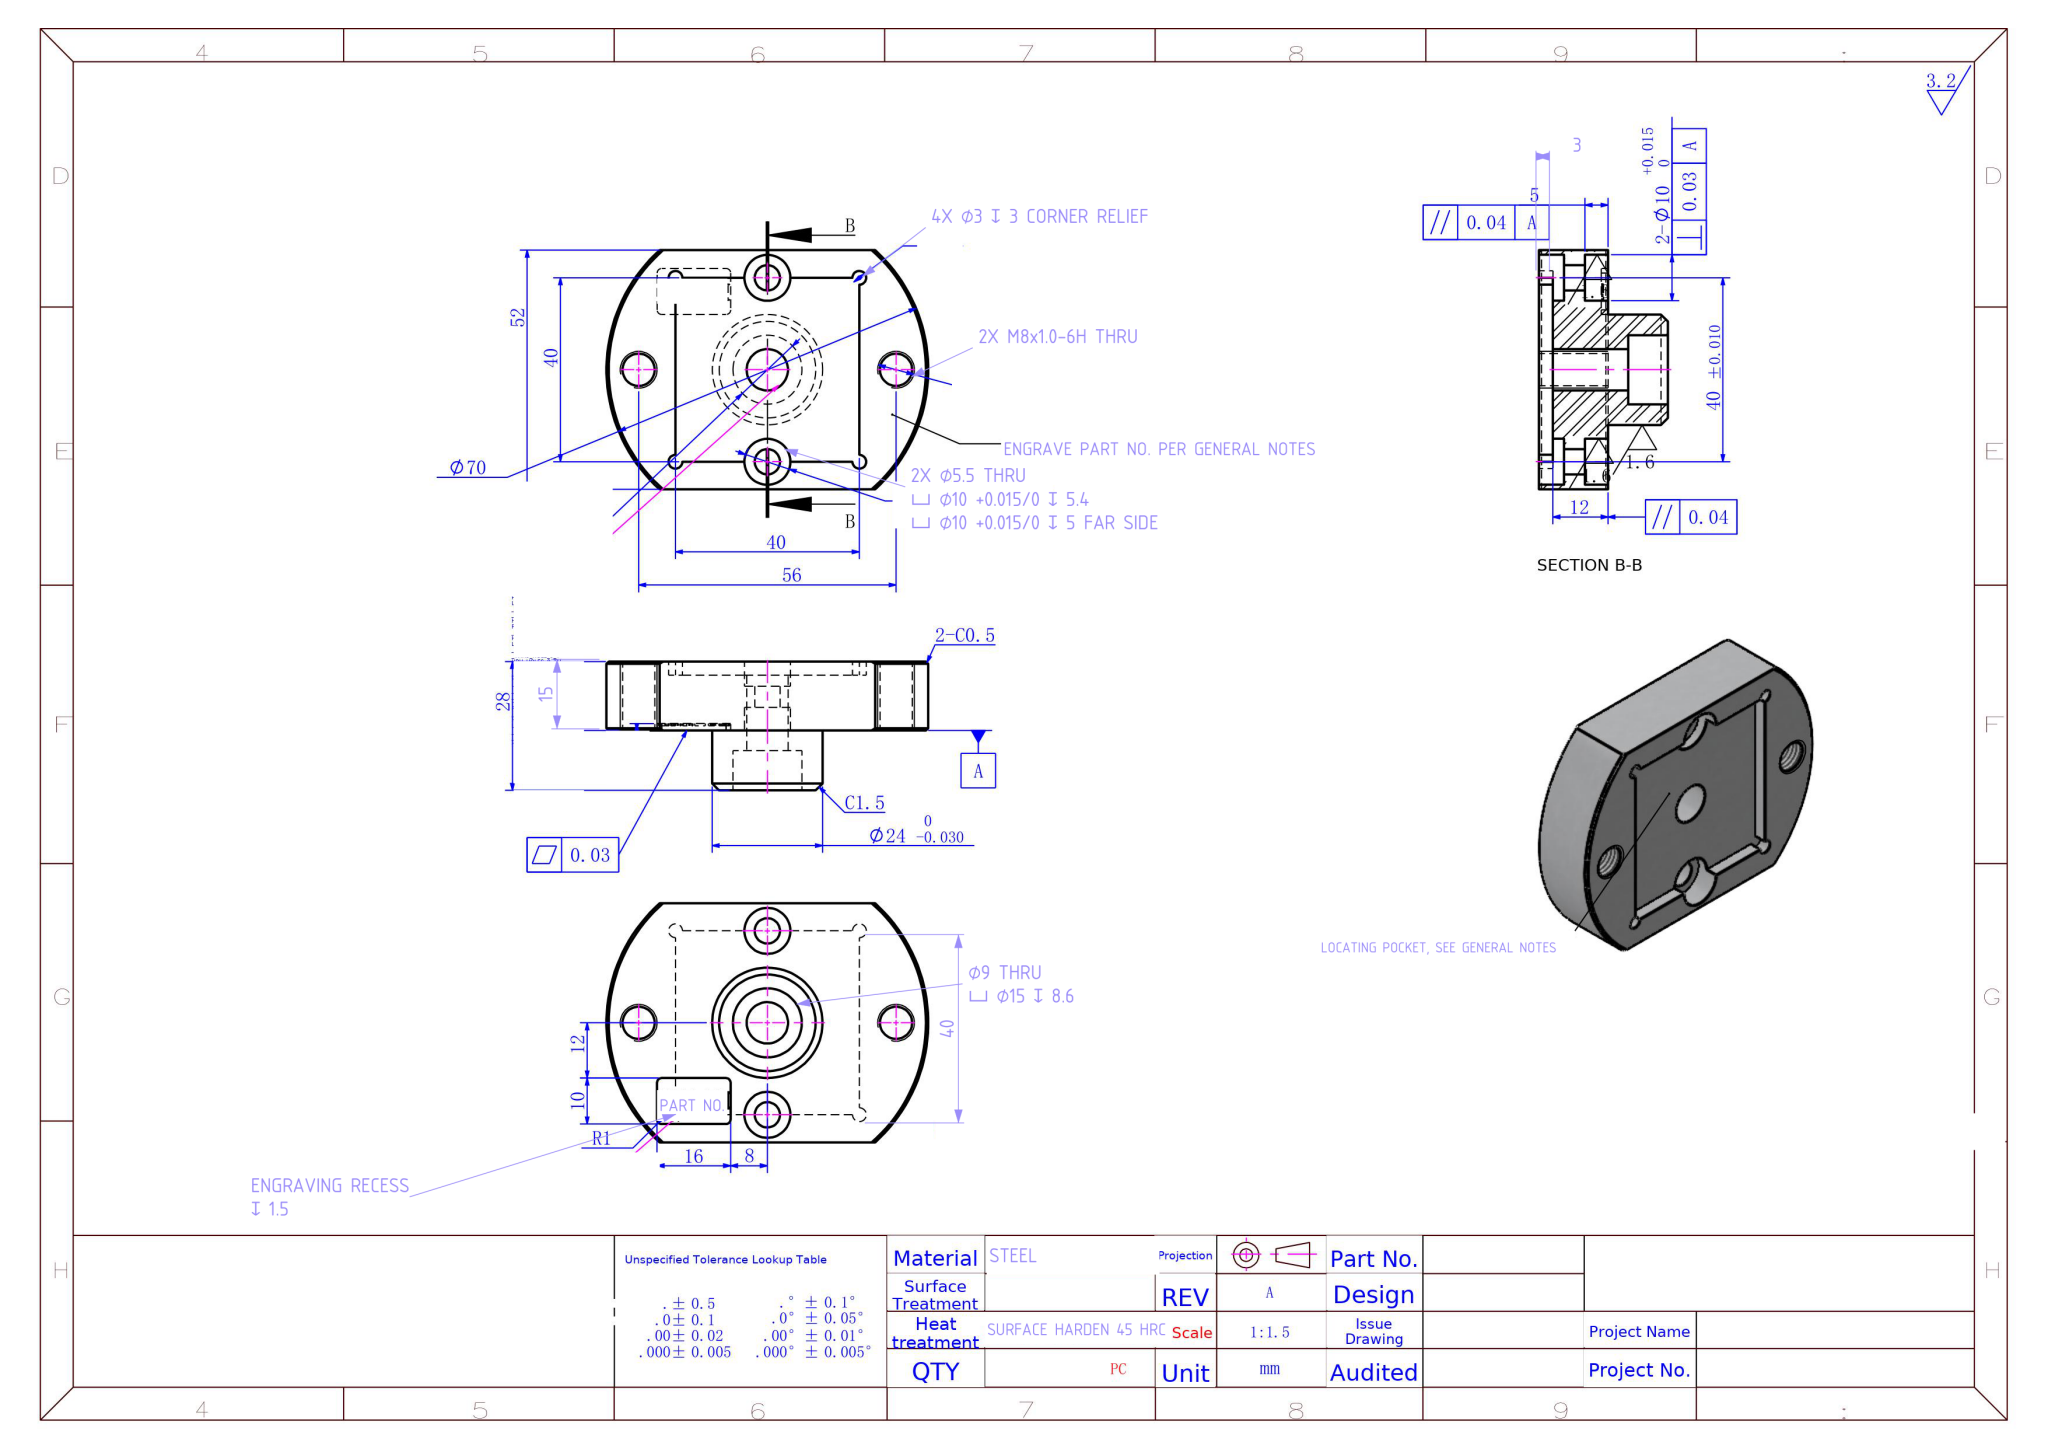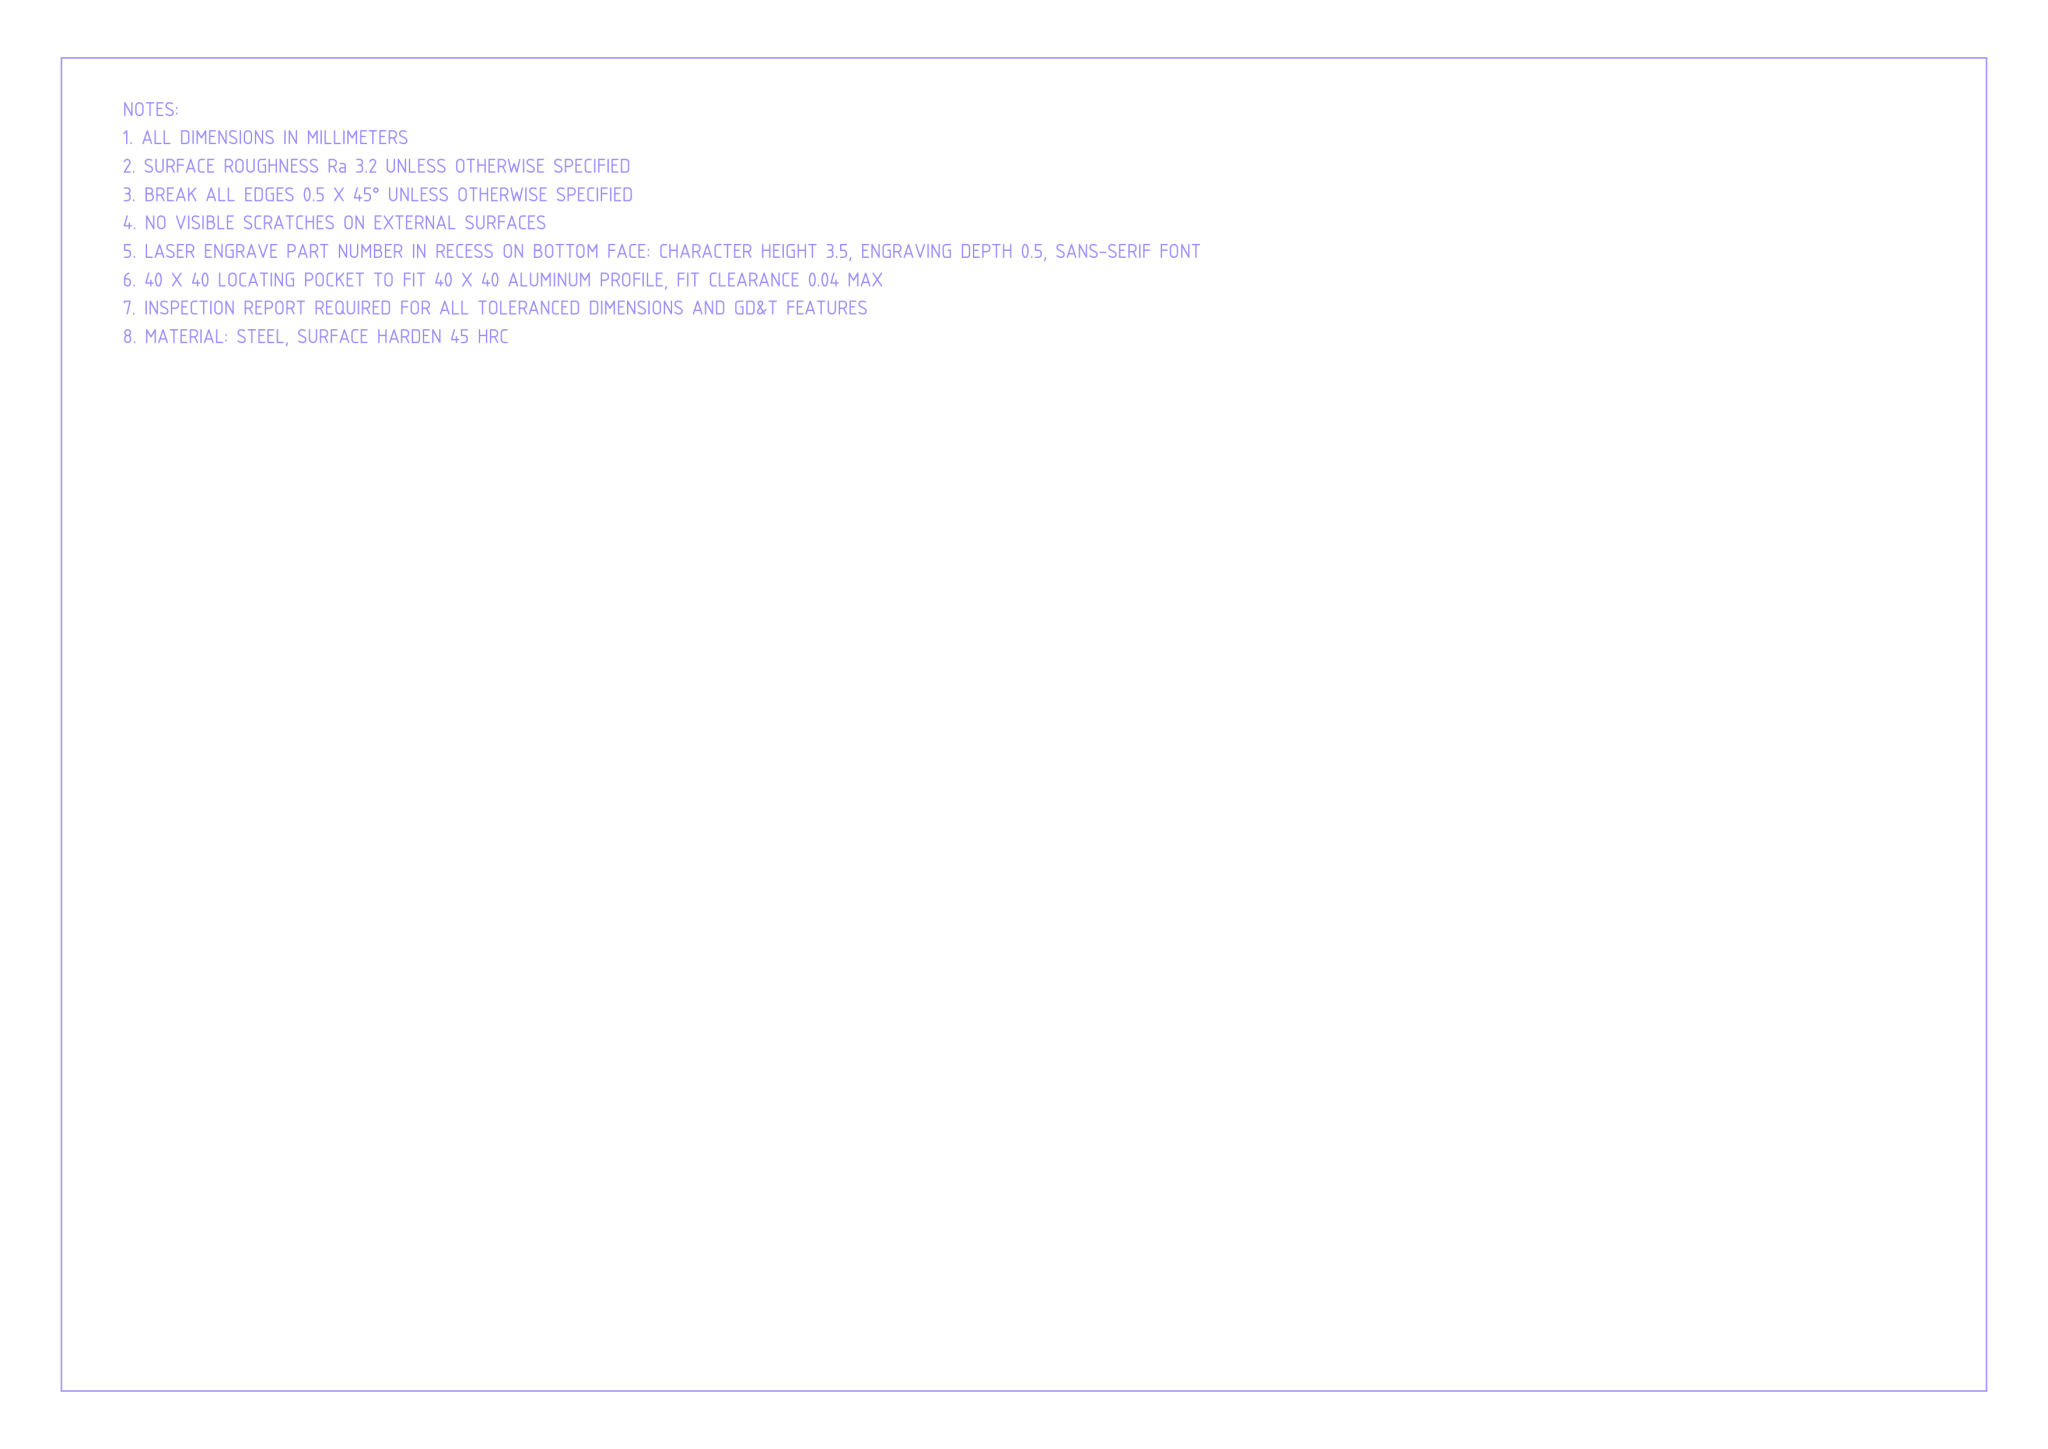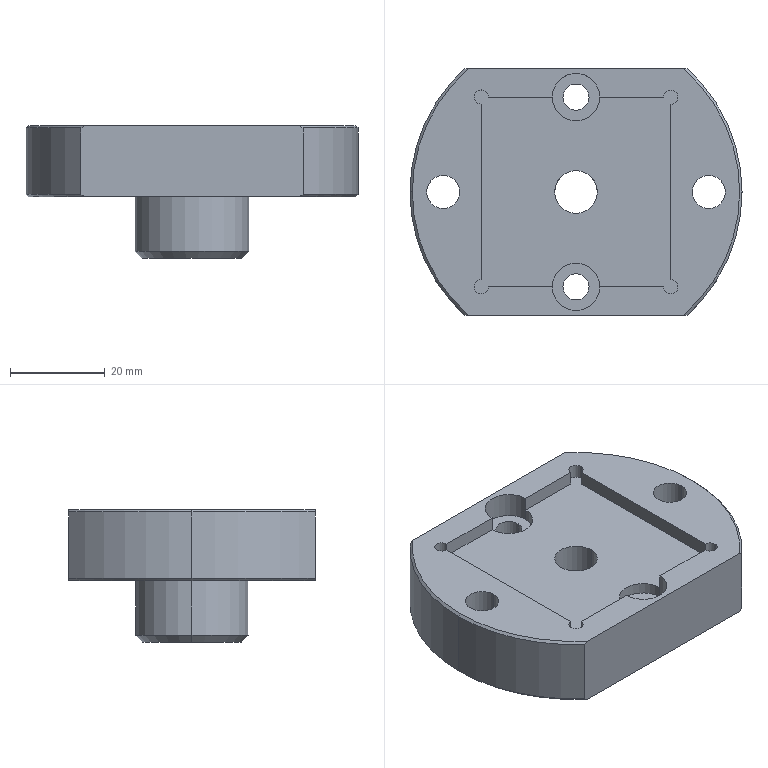Part | NX | mm | 1 solid | 187 faces | box 70 x 52 x 28 mm | volume 44387 mm3 | plane 103 | spline 41 | cylinder 35 | cone 8 | commonest cylinder face diameters 10 x8 3 x6 7 x4 5.5 x4 2 x4 70 x3 15 x2 9 x2